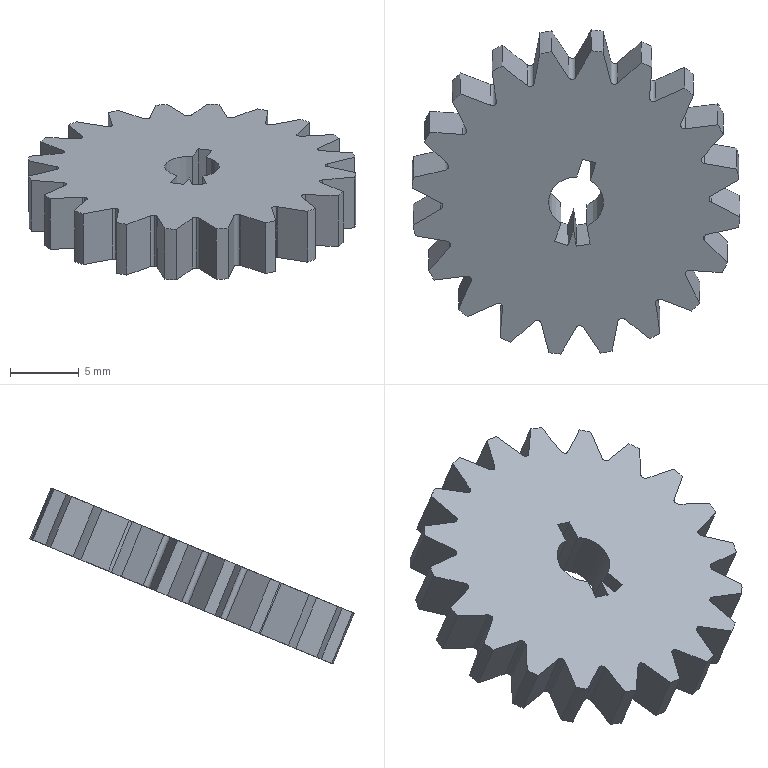Component | SolidWorks | MirrorSimple Gear-3 | 1 solid | 100 faces | volume 1442 mm3 | plane 51 | cylinder 49 | commonest cylinder face diameters 0.6 x27 24 x20 4 x2